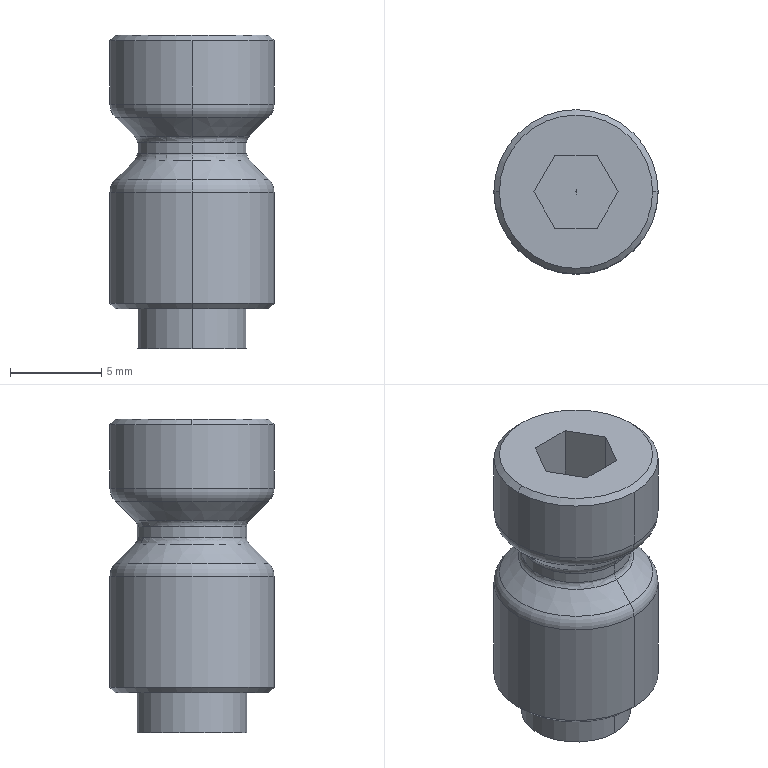Component | SolidWorks | GripperA3-2-1_SCHUNK-0303022-1 | 1 solid | 38 faces | box 9 x 9 x 17.2 mm | volume 756 mm3 | cylinder 10 | cone 10 | plane 10 | torus 8 | commonest cylinder face diameters 9 x4 6 x4 3.242 x2 | material 1.231 (40CrMnMoS8-6)
STEP:
#1=COLOUR_RGB('',0.7922,0.8196,0.9333);
#2=FILL_AREA_STYLE_COLOUR('',#1);
#3=FILL_AREA_STYLE('',(#2));
#4=SURFACE_STYLE_FILL_AREA(#3);
#5=SURFACE_SIDE_STYLE('',(#4));
#6=SURFACE_STYLE_USAGE(.BOTH.,#5);
#7=PRESENTATION_STYLE_ASSIGNMENT((#6));
#8=CARTESIAN_POINT('',(7.772,2.015,1.751));
#9=VERTEX_POINT('',#8);
#10=CARTESIAN_POINT('',(7.772,1.779,1.751));
#11=VERTEX_POINT('',#10);
#12=CARTESIAN_POINT('',(7.772,1.897,1.751));
#13=DIRECTION('',(0.,0.,1.));
#14=DIRECTION('',(0.,-1.,0.));
#15=AXIS2_PLACEMENT_3D('',#12,#13,#14);
#16=CIRCLE('',#15,0.1181);
#17=EDGE_CURVE('',#9,#11,#16,.T.);
#18=ORIENTED_EDGE('',*,*,#17,.F.);
#19=CARTESIAN_POINT('',(7.772,2.021,1.737));
#20=VERTEX_POINT('',#19);
#21=CARTESIAN_POINT('',(7.772,2.035,1.751));
#22=DIRECTION('',(1.,0.,-0.));
#23=DIRECTION('',(0.,0.,-1.));
#24=AXIS2_PLACEMENT_3D('',#21,#22,#23);
#25=CIRCLE('',#24,0.01969);
#26=EDGE_CURVE('',#9,#20,#25,.T.);
#27=ORIENTED_EDGE('',*,*,#26,.T.);
#28=CARTESIAN_POINT('',(7.772,1.773,1.737));
#29=VERTEX_POINT('',#28);
#30=CARTESIAN_POINT('',(7.772,1.897,1.737));
#31=DIRECTION('',(-0.,-0.,-1.));
#32=DIRECTION('',(0.,1.,0.));
#33=AXIS2_PLACEMENT_3D('',#30,#31,#32);
#34=CIRCLE('',#33,0.1239);
#35=EDGE_CURVE('',#29,#20,#34,.T.);
#36=ORIENTED_EDGE('',*,*,#35,.F.);
#37=CARTESIAN_POINT('',(7.772,1.759,1.751));
#38=DIRECTION('',(-1.,-0.,0.));
#39=DIRECTION('',(0.,0.,1.));
#40=AXIS2_PLACEMENT_3D('',#37,#38,#39);
#41=CIRCLE('',#40,0.01969);
#42=EDGE_CURVE('',#11,#29,#41,.T.);
#43=ORIENTED_EDGE('',*,*,#42,.F.);
#44=EDGE_LOOP('',(#18,#27,#36,#43));
#45=FACE_OUTER_BOUND('',#44,.T.);
#46=CARTESIAN_POINT('',(7.772,1.897,1.751));
#47=DIRECTION('',(0.,0.,1.));
#48=DIRECTION('',(-0.,-1.,0.));
#49=AXIS2_PLACEMENT_3D('',#46,#47,#48);
#50=TOROIDAL_SURFACE('',#49,0.1378,0.01969);
#51=ADVANCED_FACE('',(#45),#50,.F.);
#52=CARTESIAN_POINT('',(7.772,2.021,1.788));
#53=VERTEX_POINT('',#52);
#54=CARTESIAN_POINT('',(7.772,1.773,1.788));
#55=VERTEX_POINT('',#54);
#56=CARTESIAN_POINT('',(7.772,1.897,1.788));
#57=DIRECTION('',(0.,0.,1.));
#58=DIRECTION('',(0.,-1.,0.));
#59=AXIS2_PLACEMENT_3D('',#56,#57,#58);
#60=CIRCLE('',#59,0.1239);
#61=EDGE_CURVE('',#53,#55,#60,.T.);
#62=ORIENTED_EDGE('',*,*,#61,.F.);
#63=CARTESIAN_POINT('',(7.772,2.015,1.774));
#64=VERTEX_POINT('',#63);
#65=CARTESIAN_POINT('',(7.772,2.035,1.774));
#66=DIRECTION('',(1.,0.,-0.));
#67=DIRECTION('',(0.,0.,-1.));
#68=AXIS2_PLACEMENT_3D('',#65,#66,#67);
#69=CIRCLE('',#68,0.01969);
#70=EDGE_CURVE('',#53,#64,#69,.T.);
#71=ORIENTED_EDGE('',*,*,#70,.T.);
#72=CARTESIAN_POINT('',(7.772,1.779,1.774));
#73=VERTEX_POINT('',#72);
#74=CARTESIAN_POINT('',(7.772,1.897,1.774));
#75=DIRECTION('',(-0.,-0.,-1.));
#76=DIRECTION('',(0.,-1.,0.));
#77=AXIS2_PLACEMENT_3D('',#74,#75,#76);
#78=CIRCLE('',#77,0.1181);
#79=EDGE_CURVE('',#73,#64,#78,.T.);
#80=ORIENTED_EDGE('',*,*,#79,.F.);
#81=CARTESIAN_POINT('',(7.772,1.759,1.774));
#82=DIRECTION('',(-1.,-0.,0.));
#83=DIRECTION('',(0.,0.,1.));
#84=AXIS2_PLACEMENT_3D('',#81,#82,#83);
#85=CIRCLE('',#84,0.01969);
#86=EDGE_CURVE('',#55,#73,#85,.T.);
#87=ORIENTED_EDGE('',*,*,#86,.F.);
#88=EDGE_LOOP('',(#62,#71,#80,#87));
#89=FACE_OUTER_BOUND('',#88,.T.);
#90=CARTESIAN_POINT('',(7.772,1.897,1.774));
#91=DIRECTION('',(0.,0.,1.));
#92=DIRECTION('',(-0.,-1.,0.));
#93=AXIS2_PLACEMENT_3D('',#90,#91,#92);
#94=TOROIDAL_SURFACE('',#93,0.1378,0.01969);
#95=ADVANCED_FACE('',(#89),#94,.F.);
#96=CARTESIAN_POINT('',(7.772,2.074,1.668));
#97=VERTEX_POINT('',#96);
#98=CARTESIAN_POINT('',(7.772,1.72,1.668));
#99=VERTEX_POINT('',#98);
#100=CARTESIAN_POINT('',(7.772,1.897,1.668));
#101=DIRECTION('',(-0.,-0.,-1.));
#102=DIRECTION('',(-0.,-1.,0.));
#103=AXIS2_PLACEMENT_3D('',#100,#101,#102);
#104=CIRCLE('',#103,0.1772);
#105=EDGE_CURVE('',#97,#99,#104,.T.);
#106=ORIENTED_EDGE('',*,*,#105,.F.);
#107=CARTESIAN_POINT('',(7.772,2.063,1.695));
#108=VERTEX_POINT('',#107);
#109=CARTESIAN_POINT('',(7.772,2.035,1.668));
#110=DIRECTION('',(1.,0.,-0.));
#111=DIRECTION('',(0.,0.,-1.));
#112=AXIS2_PLACEMENT_3D('',#109,#110,#111);
#113=CIRCLE('',#112,0.03937);
#114=EDGE_CURVE('',#97,#108,#113,.T.);
#115=ORIENTED_EDGE('',*,*,#114,.T.);
#116=CARTESIAN_POINT('',(7.772,1.732,1.695));
#117=VERTEX_POINT('',#116);
#118=CARTESIAN_POINT('',(7.772,1.897,1.695));
#119=DIRECTION('',(0.,0.,1.));
#120=DIRECTION('',(0.,-1.,0.));
#121=AXIS2_PLACEMENT_3D('',#118,#119,#120);
#122=CIRCLE('',#121,0.1656);
#123=EDGE_CURVE('',#117,#108,#122,.T.);
#124=ORIENTED_EDGE('',*,*,#123,.F.);
#125=CARTESIAN_POINT('',(7.772,1.759,1.668));
#126=DIRECTION('',(-1.,-0.,0.));
#127=DIRECTION('',(0.,0.,1.));
#128=AXIS2_PLACEMENT_3D('',#125,#126,#127);
#129=CIRCLE('',#128,0.03937);
#130=EDGE_CURVE('',#99,#117,#129,.T.);
#131=ORIENTED_EDGE('',*,*,#130,.F.);
#132=EDGE_LOOP('',(#106,#115,#124,#131));
#133=FACE_OUTER_BOUND('',#132,.T.);
#134=CARTESIAN_POINT('',(7.772,1.897,1.668));
#135=DIRECTION('',(0.,0.,1.));
#136=DIRECTION('',(-0.,-1.,0.));
#137=AXIS2_PLACEMENT_3D('',#134,#135,#136);
#138=TOROIDAL_SURFACE('',#137,0.1378,0.03937);
#139=ADVANCED_FACE('',(#133),#138,.T.);
#140=CARTESIAN_POINT('',(7.772,1.72,1.858));
#141=VERTEX_POINT('',#140);
#142=CARTESIAN_POINT('',(7.772,2.074,1.858));
#143=VERTEX_POINT('',#142);
#144=CARTESIAN_POINT('',(7.772,1.897,1.858));
#145=DIRECTION('',(0.,0.,1.));
#146=DIRECTION('',(0.,1.,-0.));
#147=AXIS2_PLACEMENT_3D('',#144,#145,#146);
#148=CIRCLE('',#147,0.1772);
#149=EDGE_CURVE('',#141,#143,#148,.T.);
#150=ORIENTED_EDGE('',*,*,#149,.F.);
#151=CARTESIAN_POINT('',(7.772,1.732,1.83));
#152=VERTEX_POINT('',#151);
#153=CARTESIAN_POINT('',(7.772,1.759,1.858));
#154=DIRECTION('',(1.,0.,-0.));
#155=DIRECTION('',(0.,1.,0.));
#156=AXIS2_PLACEMENT_3D('',#153,#154,#155);
#157=CIRCLE('',#156,0.03937);
#158=EDGE_CURVE('',#141,#152,#157,.T.);
#159=ORIENTED_EDGE('',*,*,#158,.T.);
#160=CARTESIAN_POINT('',(7.772,2.063,1.83));
#161=VERTEX_POINT('',#160);
#162=CARTESIAN_POINT('',(7.772,1.897,1.83));
#163=DIRECTION('',(-0.,-0.,-1.));
#164=DIRECTION('',(0.,1.,-0.));
#165=AXIS2_PLACEMENT_3D('',#162,#163,#164);
#166=CIRCLE('',#165,0.1656);
#167=EDGE_CURVE('',#161,#152,#166,.T.);
#168=ORIENTED_EDGE('',*,*,#167,.F.);
#169=CARTESIAN_POINT('',(7.772,2.035,1.858));
#170=DIRECTION('',(-1.,-0.,0.));
#171=DIRECTION('',(0.,0.,1.));
#172=AXIS2_PLACEMENT_3D('',#169,#170,#171);
#173=CIRCLE('',#172,0.03937);
#174=EDGE_CURVE('',#143,#161,#173,.T.);
#175=ORIENTED_EDGE('',*,*,#174,.F.);
#176=EDGE_LOOP('',(#150,#159,#168,#175));
#177=FACE_OUTER_BOUND('',#176,.T.);
#178=CARTESIAN_POINT('',(7.772,1.897,1.858));
#179=DIRECTION('',(-0.,-0.,-1.));
#180=DIRECTION('',(0.,1.,-0.));
#181=AXIS2_PLACEMENT_3D('',#178,#179,#180);
#182=TOROIDAL_SURFACE('',#181,0.1378,0.03937);
#183=ADVANCED_FACE('',(#177),#182,.T.);
#184=CARTESIAN_POINT('',(7.95,1.897,1.995));
#185=VERTEX_POINT('',#184);
#186=CARTESIAN_POINT('',(7.772,1.72,1.995));
#187=VERTEX_POINT('',#186);
#188=CARTESIAN_POINT('',(7.772,1.897,1.995));
#189=DIRECTION('',(-0.,-0.,-1.));
#190=DIRECTION('',(0.,1.,-0.));
#191=AXIS2_PLACEMENT_3D('',#188,#189,#190);
#192=CIRCLE('',#191,0.1772);
#193=EDGE_CURVE('',#185,#187,#192,.T.);
#194=ORIENTED_EDGE('',*,*,#193,.T.);
#195=CARTESIAN_POINT('',(7.772,1.72,2.007));
#196=DIRECTION('',(-0.,-0.,-1.));
#197=VECTOR('',#196,39.37);
#198=LINE('',#195,#197);
#199=EDGE_CURVE('',#187,#141,#198,.T.);
#200=ORIENTED_EDGE('',*,*,#199,.T.);
#201=ORIENTED_EDGE('',*,*,#149,.T.);
#202=CARTESIAN_POINT('',(7.772,2.074,1.995));
#203=VERTEX_POINT('',#202);
#204=CARTESIAN_POINT('',(7.772,2.074,2.007));
#205=DIRECTION('',(-0.,-0.,-1.));
#206=VECTOR('',#205,39.37);
#207=LINE('',#204,#206);
#208=EDGE_CURVE('',#203,#143,#207,.T.);
#209=ORIENTED_EDGE('',*,*,#208,.F.);
#210=CARTESIAN_POINT('',(7.772,1.897,1.995));
#211=DIRECTION('',(-0.,-0.,-1.));
#212=DIRECTION('',(0.,1.,-0.));
#213=AXIS2_PLACEMENT_3D('',#210,#211,#212);
#214=CIRCLE('',#213,0.1772);
#215=EDGE_CURVE('',#203,#185,#214,.T.);
#216=ORIENTED_EDGE('',*,*,#215,.T.);
#217=EDGE_LOOP('',(#194,#200,#201,#209,#216));
#218=FACE_OUTER_BOUND('',#217,.T.);
#219=CARTESIAN_POINT('',(7.772,1.897,2.007));
#220=DIRECTION('',(-0.,-0.,-1.));
#221=DIRECTION('',(0.,1.,-0.));
#222=AXIS2_PLACEMENT_3D('',#219,#220,#221);
#223=CYLINDRICAL_SURFACE('',#222,0.1772);
#224=ADVANCED_FACE('',(#218),#223,.T.);
#225=CARTESIAN_POINT('',(7.607,1.897,2.007));
#226=VERTEX_POINT('',#225);
#227=CARTESIAN_POINT('',(7.938,1.897,2.007));
#228=VERTEX_POINT('',#227);
#229=CARTESIAN_POINT('',(7.772,1.897,2.007));
#230=DIRECTION('',(-0.,-0.,-1.));
#231=DIRECTION('',(-1.,-0.,0.));
#232=AXIS2_PLACEMENT_3D('',#229,#230,#231);
#233=CIRCLE('',#232,0.1654);
#234=EDGE_CURVE('',#226,#228,#233,.T.);
#235=ORIENTED_EDGE('',*,*,#234,.T.);
#236=CARTESIAN_POINT('',(7.95,1.897,1.995));
#237=DIRECTION('',(0.7071,0.,-0.7071));
#238=VECTOR('',#237,39.37);
#239=LINE('',#236,#238);
#240=EDGE_CURVE('',#228,#185,#239,.T.);
#241=ORIENTED_EDGE('',*,*,#240,.T.);
#242=ORIENTED_EDGE('',*,*,#215,.F.);
#243=CARTESIAN_POINT('',(7.595,1.897,1.995));
#244=VERTEX_POINT('',#243);
#245=CARTESIAN_POINT('',(7.772,1.897,1.995));
#246=DIRECTION('',(-0.,-0.,-1.));
#247=DIRECTION('',(0.,1.,-0.));
#248=AXIS2_PLACEMENT_3D('',#245,#246,#247);
#249=CIRCLE('',#248,0.1772);
#250=EDGE_CURVE('',#244,#203,#249,.T.);
#251=ORIENTED_EDGE('',*,*,#250,.F.);
#252=CARTESIAN_POINT('',(7.595,1.897,1.995));
#253=DIRECTION('',(-0.7071,-0.,-0.7071));
#254=VECTOR('',#253,39.37);
#255=LINE('',#252,#254);
#256=EDGE_CURVE('',#226,#244,#255,.T.);
#257=ORIENTED_EDGE('',*,*,#256,.F.);
#258=EDGE_LOOP('',(#235,#241,#242,#251,#257));
#259=FACE_OUTER_BOUND('',#258,.T.);
#260=CARTESIAN_POINT('',(7.772,1.897,1.995));
#261=DIRECTION('',(-0.,-0.,-1.));
#262=DIRECTION('',(-1.,-0.,0.));
#263=AXIS2_PLACEMENT_3D('',#260,#261,#262);
#264=CONICAL_SURFACE('',#263,0.1772,0.7854);
#265=ADVANCED_FACE('',(#259),#264,.T.);
#266=CARTESIAN_POINT('',(7.772,1.897,1.788));
#267=DIRECTION('',(0.,0.,1.));
#268=DIRECTION('',(0.,-1.,0.));
#269=AXIS2_PLACEMENT_3D('',#266,#267,#268);
#270=CIRCLE('',#269,0.1239);
#271=EDGE_CURVE('',#55,#53,#270,.T.);
#272=ORIENTED_EDGE('',*,*,#271,.T.);
#273=CARTESIAN_POINT('',(7.772,2.103,1.87));
#274=DIRECTION('',(0.,0.7071,0.7071));
#275=VECTOR('',#274,39.37);
#276=LINE('',#273,#275);
#277=EDGE_CURVE('',#53,#161,#276,.T.);
#278=ORIENTED_EDGE('',*,*,#277,.T.);
#279=ORIENTED_EDGE('',*,*,#167,.T.);
#280=CARTESIAN_POINT('',(7.772,1.691,1.87));
#281=DIRECTION('',(0.,-0.7071,0.7071));
#282=VECTOR('',#281,39.37);
#283=LINE('',#280,#282);
#284=EDGE_CURVE('',#55,#152,#283,.T.);
#285=ORIENTED_EDGE('',*,*,#284,.F.);
#286=EDGE_LOOP('',(#272,#278,#279,#285));
#287=FACE_OUTER_BOUND('',#286,.T.);
#288=CARTESIAN_POINT('',(7.772,1.897,1.87));
#289=DIRECTION('',(0.,0.,1.));
#290=DIRECTION('',(0.,-1.,0.));
#291=AXIS2_PLACEMENT_3D('',#288,#289,#290);
#292=CONICAL_SURFACE('',#291,0.2058,0.7854);
#293=ADVANCED_FACE('',(#287),#292,.T.);
#294=CARTESIAN_POINT('',(7.772,1.897,1.751));
#295=DIRECTION('',(0.,0.,1.));
#296=DIRECTION('',(0.,-1.,0.));
#297=AXIS2_PLACEMENT_3D('',#294,#295,#296);
#298=CIRCLE('',#297,0.1181);
#299=EDGE_CURVE('',#11,#9,#298,.T.);
#300=ORIENTED_EDGE('',*,*,#299,.T.);
#301=CARTESIAN_POINT('',(7.772,2.015,1.772));
#302=DIRECTION('',(0.,0.,1.));
#303=VECTOR('',#302,39.37);
#304=LINE('',#301,#303);
#305=EDGE_CURVE('',#9,#64,#304,.T.);
#306=ORIENTED_EDGE('',*,*,#305,.T.);
#307=CARTESIAN_POINT('',(7.772,1.897,1.774));
#308=DIRECTION('',(-0.,-0.,-1.));
#309=DIRECTION('',(0.,-1.,0.));
#310=AXIS2_PLACEMENT_3D('',#307,#308,#309);
#311=CIRCLE('',#310,0.1181);
#312=EDGE_CURVE('',#64,#73,#311,.T.);
#313=ORIENTED_EDGE('',*,*,#312,.T.);
#314=CARTESIAN_POINT('',(7.772,1.779,1.772));
#315=DIRECTION('',(0.,0.,1.));
#316=VECTOR('',#315,39.37);
#317=LINE('',#314,#316);
#318=EDGE_CURVE('',#11,#73,#317,.T.);
#319=ORIENTED_EDGE('',*,*,#318,.F.);
#320=EDGE_LOOP('',(#300,#306,#313,#319));
#321=FACE_OUTER_BOUND('',#320,.T.);
#322=CARTESIAN_POINT('',(7.772,1.897,1.772));
#323=DIRECTION('',(0.,0.,1.));
#324=DIRECTION('',(0.,-1.,0.));
#325=AXIS2_PLACEMENT_3D('',#322,#323,#324);
#326=CYLINDRICAL_SURFACE('',#325,0.1181);
#327=ADVANCED_FACE('',(#321),#326,.T.);
#328=CARTESIAN_POINT('',(7.772,1.897,1.737));
#329=DIRECTION('',(-0.,-0.,-1.));
#330=DIRECTION('',(0.,1.,0.));
#331=AXIS2_PLACEMENT_3D('',#328,#329,#330);
#332=CIRCLE('',#331,0.1239);
#333=EDGE_CURVE('',#20,#29,#332,.T.);
#334=ORIENTED_EDGE('',*,*,#333,.T.);
#335=CARTESIAN_POINT('',(7.772,1.779,1.743));
#336=DIRECTION('',(0.,-0.7071,-0.7071));
#337=VECTOR('',#336,39.37);
#338=LINE('',#335,#337);
#339=EDGE_CURVE('',#29,#117,#338,.T.);
#340=ORIENTED_EDGE('',*,*,#339,.T.);
#341=ORIENTED_EDGE('',*,*,#123,.T.);
#342=CARTESIAN_POINT('',(7.772,2.015,1.743));
#343=DIRECTION('',(-0.,0.7071,-0.7071));
#344=VECTOR('',#343,39.37);
#345=LINE('',#342,#344);
#346=EDGE_CURVE('',#20,#108,#345,.T.);
#347=ORIENTED_EDGE('',*,*,#346,.F.);
#348=EDGE_LOOP('',(#334,#340,#341,#347));
#349=FACE_OUTER_BOUND('',#348,.T.);
#350=CARTESIAN_POINT('',(7.772,1.897,1.743));
#351=DIRECTION('',(-0.,-0.,-1.));
#352=DIRECTION('',(0.,1.,0.));
#353=AXIS2_PLACEMENT_3D('',#350,#351,#352);
#354=CONICAL_SURFACE('',#353,0.1181,0.7854);
#355=ADVANCED_FACE('',(#349),#354,.T.);
#356=CARTESIAN_POINT('',(7.772,1.732,1.416));
#357=VERTEX_POINT('',#356);
#358=CARTESIAN_POINT('',(7.772,2.063,1.416));
#359=VERTEX_POINT('',#358);
#360=CARTESIAN_POINT('',(7.772,1.897,1.416));
#361=DIRECTION('',(0.,0.,1.));
#362=DIRECTION('',(0.,-1.,0.));
#363=AXIS2_PLACEMENT_3D('',#360,#361,#362);
#364=CIRCLE('',#363,0.1654);
#365=EDGE_CURVE('',#357,#359,#364,.T.);
#366=ORIENTED_EDGE('',*,*,#365,.T.);
#367=CARTESIAN_POINT('',(7.772,2.074,1.428));
#368=VERTEX_POINT('',#367);
#369=CARTESIAN_POINT('',(7.772,2.074,1.428));
#370=DIRECTION('',(0.,0.7071,0.7071));
#371=VECTOR('',#370,39.37);
#372=LINE('',#369,#371);
#373=EDGE_CURVE('',#359,#368,#372,.T.);
#374=ORIENTED_EDGE('',*,*,#373,.T.);
#375=CARTESIAN_POINT('',(7.772,1.72,1.428));
#376=VERTEX_POINT('',#375);
#377=CARTESIAN_POINT('',(7.772,1.897,1.428));
#378=DIRECTION('',(0.,0.,1.));
#379=DIRECTION('',(-0.,1.,-0.));
#380=AXIS2_PLACEMENT_3D('',#377,#378,#379);
#381=CIRCLE('',#380,0.1772);
#382=EDGE_CURVE('',#376,#368,#381,.T.);
#383=ORIENTED_EDGE('',*,*,#382,.F.);
#384=CARTESIAN_POINT('',(7.772,1.72,1.428));
#385=DIRECTION('',(0.,-0.7071,0.7071));
#386=VECTOR('',#385,39.37);
#387=LINE('',#384,#386);
#388=EDGE_CURVE('',#357,#376,#387,.T.);
#389=ORIENTED_EDGE('',*,*,#388,.F.);
#390=EDGE_LOOP('',(#366,#374,#383,#389));
#391=FACE_OUTER_BOUND('',#390,.T.);
#392=CARTESIAN_POINT('',(7.772,1.897,1.428));
#393=DIRECTION('',(0.,0.,1.));
#394=DIRECTION('',(0.,-1.,0.));
#395=AXIS2_PLACEMENT_3D('',#392,#393,#394);
#396=CONICAL_SURFACE('',#395,0.1772,0.7854);
#397=ADVANCED_FACE('',(#391),#396,.T.);
#398=CARTESIAN_POINT('',(7.772,2.015,1.416));
#399=VERTEX_POINT('',#398);
#400=CARTESIAN_POINT('',(7.772,1.779,1.416));
#401=VERTEX_POINT('',#400);
#402=CARTESIAN_POINT('',(7.772,1.897,1.416));
#403=DIRECTION('',(-0.,-0.,-1.));
#404=DIRECTION('',(0.,1.,0.));
#405=AXIS2_PLACEMENT_3D('',#402,#403,#404);
#406=CIRCLE('',#405,0.1181);
#407=EDGE_CURVE('',#399,#401,#406,.T.);
#408=ORIENTED_EDGE('',*,*,#407,.T.);
#409=CARTESIAN_POINT('',(7.772,1.779,1.33));
#410=VERTEX_POINT('',#409);
#411=CARTESIAN_POINT('',(7.772,1.779,2.007));
#412=DIRECTION('',(-0.,-0.,-1.));
#413=VECTOR('',#412,39.37);
#414=LINE('',#411,#413);
#415=EDGE_CURVE('',#401,#410,#414,.T.);
#416=ORIENTED_EDGE('',*,*,#415,.T.);
#417=CARTESIAN_POINT('',(7.772,2.015,1.33));
#418=VERTEX_POINT('',#417);
#419=CARTESIAN_POINT('',(7.772,1.897,1.33));
#420=DIRECTION('',(0.,0.,1.));
#421=DIRECTION('',(0.,1.,0.));
#422=AXIS2_PLACEMENT_3D('',#419,#420,#421);
#423=CIRCLE('',#422,0.1181);
#424=EDGE_CURVE('',#410,#418,#423,.T.);
#425=ORIENTED_EDGE('',*,*,#424,.T.);
#426=CARTESIAN_POINT('',(7.772,2.015,2.007));
#427=DIRECTION('',(-0.,-0.,-1.));
#428=VECTOR('',#427,39.37);
#429=LINE('',#426,#428);
#430=EDGE_CURVE('',#399,#418,#429,.T.);
#431=ORIENTED_EDGE('',*,*,#430,.F.);
#432=EDGE_LOOP('',(#408,#416,#425,#431));
#433=FACE_OUTER_BOUND('',#432,.T.);
#434=CARTESIAN_POINT('',(7.772,1.897,2.007));
#435=DIRECTION('',(-0.,-0.,-1.));
#436=DIRECTION('',(0.,1.,0.));
#437=AXIS2_PLACEMENT_3D('',#434,#435,#436);
#438=CYLINDRICAL_SURFACE('',#437,0.1181);
#439=ADVANCED_FACE('',(#433),#438,.T.);
#440=CARTESIAN_POINT('',(7.772,1.833,1.772));
#441=VERTEX_POINT('',#440);
#442=CARTESIAN_POINT('',(7.772,1.961,1.772));
#443=VERTEX_POINT('',#442);
#444=CARTESIAN_POINT('',(7.772,1.897,1.772));
#445=DIRECTION('',(-0.,-0.,-1.));
#446=DIRECTION('',(0.,1.,0.));
#447=AXIS2_PLACEMENT_3D('',#444,#445,#446);
#448=CIRCLE('',#447,0.06382);
#449=EDGE_CURVE('',#441,#443,#448,.T.);
#450=ORIENTED_EDGE('',*,*,#449,.F.);
#451=CARTESIAN_POINT('',(7.772,1.833,1.33));
#452=VERTEX_POINT('',#451);
#453=CARTESIAN_POINT('',(7.772,1.833,2.007));
#454=DIRECTION('',(-0.,-0.,-1.));
#455=VECTOR('',#454,39.37);
#456=LINE('',#453,#455);
#457=EDGE_CURVE('',#441,#452,#456,.T.);
#458=ORIENTED_EDGE('',*,*,#457,.T.);
#459=CARTESIAN_POINT('',(7.772,1.961,1.33));
#460=VERTEX_POINT('',#459);
#461=CARTESIAN_POINT('',(7.772,1.897,1.33));
#462=DIRECTION('',(-0.,-0.,-1.));
#463=DIRECTION('',(0.,1.,0.));
#464=AXIS2_PLACEMENT_3D('',#461,#462,#463);
#465=CIRCLE('',#464,0.06382);
#466=EDGE_CURVE('',#452,#460,#465,.T.);
#467=ORIENTED_EDGE('',*,*,#466,.T.);
#468=CARTESIAN_POINT('',(7.772,1.961,2.007));
#469=DIRECTION('',(-0.,-0.,-1.));
#470=VECTOR('',#469,39.37);
#471=LINE('',#468,#470);
#472=EDGE_CURVE('',#443,#460,#471,.T.);
#473=ORIENTED_EDGE('',*,*,#472,.F.);
#474=EDGE_LOOP('',(#450,#458,#467,#473));
#475=FACE_OUTER_BOUND('',#474,.T.);
#476=CARTESIAN_POINT('',(7.772,1.897,2.007));
#477=DIRECTION('',(-0.,-0.,-1.));
#478=DIRECTION('',(0.,1.,0.));
#479=AXIS2_PLACEMENT_3D('',#476,#477,#478);
#480=CYLINDRICAL_SURFACE('',#479,0.06382);
#481=ADVANCED_FACE('',(#475),#480,.F.);
#482=ORIENTED_EDGE('',*,*,#105,.T.);
#483=CARTESIAN_POINT('',(7.772,1.72,2.007));
#484=DIRECTION('',(-0.,-0.,-1.));
#485=VECTOR('',#484,39.37);
#486=LINE('',#483,#485);
#487=EDGE_CURVE('',#99,#376,#486,.T.);
#488=ORIENTED_EDGE('',*,*,#487,.T.);
#489=ORIENTED_EDGE('',*,*,#382,.T.);
#490=CARTESIAN_POINT('',(7.772,2.074,2.007));
#491=DIRECTION('',(-0.,-0.,-1.));
#492=VECTOR('',#491,39.37);
#493=LINE('',#490,#492);
#494=EDGE_CURVE('',#97,#368,#493,.T.);
#495=ORIENTED_EDGE('',*,*,#494,.F.);
#496=EDGE_LOOP('',(#482,#488,#489,#495));
#497=FACE_OUTER_BOUND('',#496,.T.);
#498=CARTESIAN_POINT('',(7.772,1.897,2.007));
#499=DIRECTION('',(-0.,-0.,-1.));
#500=DIRECTION('',(0.,1.,-0.));
#501=AXIS2_PLACEMENT_3D('',#498,#499,#500);
#502=CYLINDRICAL_SURFACE('',#501,0.1772);
#503=ADVANCED_FACE('',(#497),#502,.T.);
#504=CARTESIAN_POINT('',(7.772,1.897,1.81));
#505=VERTEX_POINT('',#504);
#506=CARTESIAN_POINT('',(7.772,1.897,1.81));
#507=VERTEX_POINT('',#506);
#508=CARTESIAN_POINT('',(7.772,1.897,1.81));
#509=DIRECTION('',(-0.,-0.,-1.));
#510=DIRECTION('',(0.,-1.,0.));
#511=AXIS2_PLACEMENT_3D('',#508,#509,#510);
#512=CIRCLE('',#511,0.0001128);
#513=EDGE_CURVE('',#505,#507,#512,.T.);
#514=ORIENTED_EDGE('',*,*,#513,.F.);
#515=CARTESIAN_POINT('',(7.772,1.833,1.772));
#516=DIRECTION('',(0.,-0.8572,-0.515));
#517=VECTOR('',#516,39.37);
#518=LINE('',#515,#517);
#519=EDGE_CURVE('',#505,#441,#518,.T.);
#520=ORIENTED_EDGE('',*,*,#519,.T.);
#521=ORIENTED_EDGE('',*,*,#449,.T.);
#522=CARTESIAN_POINT('',(7.772,1.961,1.772));
#523=DIRECTION('',(-0.,0.8572,-0.515));
#524=VECTOR('',#523,39.37);
#525=LINE('',#522,#524);
#526=EDGE_CURVE('',#507,#443,#525,.T.);
#527=ORIENTED_EDGE('',*,*,#526,.F.);
#528=EDGE_LOOP('',(#514,#520,#521,#527));
#529=FACE_OUTER_BOUND('',#528,.T.);
#530=CARTESIAN_POINT('',(7.772,1.897,1.772));
#531=DIRECTION('',(-0.,-0.,-1.));
#532=DIRECTION('',(0.,1.,0.));
#533=AXIS2_PLACEMENT_3D('',#530,#531,#532);
#534=CONICAL_SURFACE('',#533,0.06382,1.03);
#535=ADVANCED_FACE('',(#529),#534,.F.);
#536=ORIENTED_EDGE('',*,*,#519,.F.);
#537=CARTESIAN_POINT('',(7.772,1.897,1.81));
#538=DIRECTION('',(-0.,-0.,-1.));
#539=DIRECTION('',(0.,-1.,0.));
#540=AXIS2_PLACEMENT_3D('',#537,#538,#539);
#541=CIRCLE('',#540,0.0001128);
#542=EDGE_CURVE('',#507,#505,#541,.T.);
#543=ORIENTED_EDGE('',*,*,#542,.F.);
#544=ORIENTED_EDGE('',*,*,#526,.T.);
#545=CARTESIAN_POINT('',(7.772,1.897,1.772));
#546=DIRECTION('',(-0.,-0.,-1.));
#547=DIRECTION('',(0.,1.,0.));
#548=AXIS2_PLACEMENT_3D('',#545,#546,#547);
#549=CIRCLE('',#548,0.06382);
#550=EDGE_CURVE('',#443,#441,#549,.T.);
#551=ORIENTED_EDGE('',*,*,#550,.T.);
#552=EDGE_LOOP('',(#536,#543,#544,#551));
#553=FACE_OUTER_BOUND('',#552,.T.);
#554=CARTESIAN_POINT('',(7.772,1.897,1.772));
#555=DIRECTION('',(-0.,-0.,-1.));
#556=DIRECTION('',(0.,1.,0.));
#557=AXIS2_PLACEMENT_3D('',#554,#555,#556);
#558=CONICAL_SURFACE('',#557,0.06382,1.03);
#559=ADVANCED_FACE('',(#553),#558,.F.);
#560=ORIENTED_EDGE('',*,*,#487,.F.);
#561=CARTESIAN_POINT('',(7.772,1.897,1.668));
#562=DIRECTION('',(-0.,-0.,-1.));
#563=DIRECTION('',(0.,-1.,0.));
#564=AXIS2_PLACEMENT_3D('',#561,#562,#563);
#565=CIRCLE('',#564,0.1772);
#566=EDGE_CURVE('',#99,#97,#565,.T.);
#567=ORIENTED_EDGE('',*,*,#566,.T.);
#568=ORIENTED_EDGE('',*,*,#494,.T.);
#569=CARTESIAN_POINT('',(7.772,1.897,1.428));
#570=DIRECTION('',(0.,0.,1.));
#571=DIRECTION('',(0.,1.,-0.));
#572=AXIS2_PLACEMENT_3D('',#569,#570,#571);
#573=CIRCLE('',#572,0.1772);
#574=EDGE_CURVE('',#368,#376,#573,.T.);
#575=ORIENTED_EDGE('',*,*,#574,.T.);
#576=EDGE_LOOP('',(#560,#567,#568,#575));
#577=FACE_OUTER_BOUND('',#576,.T.);
#578=CARTESIAN_POINT('',(7.772,1.897,2.007));
#579=DIRECTION('',(-0.,-0.,-1.));
#580=DIRECTION('',(0.,1.,-0.));
#581=AXIS2_PLACEMENT_3D('',#578,#579,#580);
#582=CYLINDRICAL_SURFACE('',#581,0.1772);
#583=ADVANCED_FACE('',(#577),#582,.T.);
#584=ORIENTED_EDGE('',*,*,#373,.F.);
#585=CARTESIAN_POINT('',(7.772,1.897,1.416));
#586=DIRECTION('',(0.,0.,1.));
#587=DIRECTION('',(0.,-1.,0.));
#588=AXIS2_PLACEMENT_3D('',#585,#586,#587);
#589=CIRCLE('',#588,0.1654);
#590=EDGE_CURVE('',#359,#357,#589,.T.);
#591=ORIENTED_EDGE('',*,*,#590,.T.);
#592=ORIENTED_EDGE('',*,*,#388,.T.);
#593=ORIENTED_EDGE('',*,*,#574,.F.);
#594=EDGE_LOOP('',(#584,#591,#592,#593));
#595=FACE_OUTER_BOUND('',#594,.T.);
#596=CARTESIAN_POINT('',(7.772,1.897,1.428));
#597=DIRECTION('',(0.,0.,1.));
#598=DIRECTION('',(0.,-1.,0.));
#599=AXIS2_PLACEMENT_3D('',#596,#597,#598);
#600=CONICAL_SURFACE('',#599,0.1772,0.7854);
#601=ADVANCED_FACE('',(#595),#600,.T.);
#602=ORIENTED_EDGE('',*,*,#407,.F.);
#603=CARTESIAN_POINT('',(7.772,1.897,1.416));
#604=DIRECTION('',(-0.,-0.,-1.));
#605=DIRECTION('',(0.,1.,0.));
#606=AXIS2_PLACEMENT_3D('',#603,#604,#605);
#607=CIRCLE('',#606,0.1181);
#608=EDGE_CURVE('',#401,#399,#607,.T.);
#609=ORIENTED_EDGE('',*,*,#608,.F.);
#610=EDGE_LOOP('',(#602,#609));
#611=FACE_BOUND('',#610,.T.);
#612=ORIENTED_EDGE('',*,*,#365,.F.);
#613=ORIENTED_EDGE('',*,*,#590,.F.);
#614=EDGE_LOOP('',(#612,#613));
#615=FACE_OUTER_BOUND('',#614,.T.);
#616=CARTESIAN_POINT('',(7.772,1.779,1.416));
#617=DIRECTION('',(0.,0.,1.));
#618=DIRECTION('',(0.,-1.,0.));
#619=AXIS2_PLACEMENT_3D('',#616,#617,#618);
#620=PLANE('',#619);
#621=ADVANCED_FACE('',(#611,#615),#620,.F.);
#622=ORIENTED_EDGE('',*,*,#415,.F.);
#623=ORIENTED_EDGE('',*,*,#608,.T.);
#624=ORIENTED_EDGE('',*,*,#430,.T.);
#625=CARTESIAN_POINT('',(7.772,1.897,1.33));
#626=DIRECTION('',(0.,0.,1.));
#627=DIRECTION('',(0.,1.,0.));
#628=AXIS2_PLACEMENT_3D('',#625,#626,#627);
#629=CIRCLE('',#628,0.1181);
#630=EDGE_CURVE('',#418,#410,#629,.T.);
#631=ORIENTED_EDGE('',*,*,#630,.T.);
#632=EDGE_LOOP('',(#622,#623,#624,#631));
#633=FACE_OUTER_BOUND('',#632,.T.);
#634=CARTESIAN_POINT('',(7.772,1.897,2.007));
#635=DIRECTION('',(-0.,-0.,-1.));
#636=DIRECTION('',(0.,1.,0.));
#637=AXIS2_PLACEMENT_3D('',#634,#635,#636);
#638=CYLINDRICAL_SURFACE('',#637,0.1181);
#639=ADVANCED_FACE('',(#633),#638,.T.);
#640=CARTESIAN_POINT('',(7.772,1.897,1.33));
#641=DIRECTION('',(-0.,-0.,-1.));
#642=DIRECTION('',(0.,1.,0.));
#643=AXIS2_PLACEMENT_3D('',#640,#641,#642);
#644=CIRCLE('',#643,0.06382);
#645=EDGE_CURVE('',#460,#452,#644,.T.);
#646=ORIENTED_EDGE('',*,*,#645,.F.);
#647=ORIENTED_EDGE('',*,*,#466,.F.);
#648=EDGE_LOOP('',(#646,#647));
#649=FACE_BOUND('',#648,.T.);
#650=ORIENTED_EDGE('',*,*,#630,.F.);
#651=ORIENTED_EDGE('',*,*,#424,.F.);
#652=EDGE_LOOP('',(#650,#651));
#653=FACE_OUTER_BOUND('',#652,.T.);
#654=CARTESIAN_POINT('',(7.772,1.833,1.33));
#655=DIRECTION('',(0.,0.,1.));
#656=DIRECTION('',(0.,-1.,0.));
#657=AXIS2_PLACEMENT_3D('',#654,#655,#656);
#658=PLANE('',#657);
#659=ADVANCED_FACE('',(#649,#653),#658,.F.);
#660=ORIENTED_EDGE('',*,*,#457,.F.);
#661=ORIENTED_EDGE('',*,*,#550,.F.);
#662=ORIENTED_EDGE('',*,*,#472,.T.);
#663=ORIENTED_EDGE('',*,*,#645,.T.);
#664=EDGE_LOOP('',(#660,#661,#662,#663));
#665=FACE_OUTER_BOUND('',#664,.T.);
#666=CARTESIAN_POINT('',(7.772,1.897,2.007));
#667=DIRECTION('',(-0.,-0.,-1.));
#668=DIRECTION('',(0.,1.,0.));
#669=AXIS2_PLACEMENT_3D('',#666,#667,#668);
#670=CYLINDRICAL_SURFACE('',#669,0.06382);
#671=ADVANCED_FACE('',(#665),#670,.F.);
#672=ORIENTED_EDGE('',*,*,#339,.F.);
#673=ORIENTED_EDGE('',*,*,#35,.T.);
#674=ORIENTED_EDGE('',*,*,#346,.T.);
#675=CARTESIAN_POINT('',(7.772,1.897,1.695));
#676=DIRECTION('',(0.,0.,1.));
#677=DIRECTION('',(0.,-1.,0.));
#678=AXIS2_PLACEMENT_3D('',#675,#676,#677);
#679=CIRCLE('',#678,0.1656);
#680=EDGE_CURVE('',#108,#117,#679,.T.);
#681=ORIENTED_EDGE('',*,*,#680,.T.);
#682=EDGE_LOOP('',(#672,#673,#674,#681));
#683=FACE_OUTER_BOUND('',#682,.T.);
#684=CARTESIAN_POINT('',(7.772,1.897,1.743));
#685=DIRECTION('',(-0.,-0.,-1.));
#686=DIRECTION('',(0.,1.,0.));
#687=AXIS2_PLACEMENT_3D('',#684,#685,#686);
#688=CONICAL_SURFACE('',#687,0.1181,0.7854);
#689=ADVANCED_FACE('',(#683),#688,.T.);
#690=ORIENTED_EDGE('',*,*,#305,.F.);
#691=ORIENTED_EDGE('',*,*,#17,.T.);
#692=ORIENTED_EDGE('',*,*,#318,.T.);
#693=ORIENTED_EDGE('',*,*,#79,.T.);
#694=EDGE_LOOP('',(#690,#691,#692,#693));
#695=FACE_OUTER_BOUND('',#694,.T.);
#696=CARTESIAN_POINT('',(7.772,1.897,1.772));
#697=DIRECTION('',(0.,0.,1.));
#698=DIRECTION('',(0.,-1.,0.));
#699=AXIS2_PLACEMENT_3D('',#696,#697,#698);
#700=CYLINDRICAL_SURFACE('',#699,0.1181);
#701=ADVANCED_FACE('',(#695),#700,.T.);
#702=ORIENTED_EDGE('',*,*,#277,.F.);
#703=ORIENTED_EDGE('',*,*,#61,.T.);
#704=ORIENTED_EDGE('',*,*,#284,.T.);
#705=CARTESIAN_POINT('',(7.772,1.897,1.83));
#706=DIRECTION('',(-0.,-0.,-1.));
#707=DIRECTION('',(0.,1.,-0.));
#708=AXIS2_PLACEMENT_3D('',#705,#706,#707);
#709=CIRCLE('',#708,0.1656);
#710=EDGE_CURVE('',#152,#161,#709,.T.);
#711=ORIENTED_EDGE('',*,*,#710,.T.);
#712=EDGE_LOOP('',(#702,#703,#704,#711));
#713=FACE_OUTER_BOUND('',#712,.T.);
#714=CARTESIAN_POINT('',(7.772,1.897,1.87));
#715=DIRECTION('',(0.,0.,1.));
#716=DIRECTION('',(0.,-1.,0.));
#717=AXIS2_PLACEMENT_3D('',#714,#715,#716);
#718=CONICAL_SURFACE('',#717,0.2058,0.7854);
#719=ADVANCED_FACE('',(#713),#718,.T.);
#720=CARTESIAN_POINT('',(7.682,1.897,2.007));
#721=VERTEX_POINT('',#720);
#722=CARTESIAN_POINT('',(7.727,1.818,2.007));
#723=VERTEX_POINT('',#722);
#724=CARTESIAN_POINT('',(7.682,1.897,2.007));
#725=DIRECTION('',(0.5,-0.866,0.));
#726=VECTOR('',#725,39.37);
#727=LINE('',#724,#726);
#728=EDGE_CURVE('',#721,#723,#727,.T.);
#729=ORIENTED_EDGE('',*,*,#728,.F.);
#730=CARTESIAN_POINT('',(7.727,1.976,2.007));
#731=VERTEX_POINT('',#730);
#732=CARTESIAN_POINT('',(7.727,1.976,2.007));
#733=DIRECTION('',(-0.5,-0.866,0.));
#734=VECTOR('',#733,39.37);
#735=LINE('',#732,#734);
#736=EDGE_CURVE('',#731,#721,#735,.T.);
#737=ORIENTED_EDGE('',*,*,#736,.F.);
#738=CARTESIAN_POINT('',(7.818,1.976,2.007));
#739=VERTEX_POINT('',#738);
#740=CARTESIAN_POINT('',(7.818,1.976,2.007));
#741=DIRECTION('',(-1.,-0.,0.));
#742=VECTOR('',#741,39.37);
#743=LINE('',#740,#742);
#744=EDGE_CURVE('',#739,#731,#743,.T.);
#745=ORIENTED_EDGE('',*,*,#744,.F.);
#746=CARTESIAN_POINT('',(7.863,1.897,2.007));
#747=VERTEX_POINT('',#746);
#748=CARTESIAN_POINT('',(7.863,1.897,2.007));
#749=DIRECTION('',(-0.5,0.866,-0.));
#750=VECTOR('',#749,39.37);
#751=LINE('',#748,#750);
#752=EDGE_CURVE('',#747,#739,#751,.T.);
#753=ORIENTED_EDGE('',*,*,#752,.F.);
#754=CARTESIAN_POINT('',(7.818,1.818,2.007));
#755=VERTEX_POINT('',#754);
#756=CARTESIAN_POINT('',(7.818,1.818,2.007));
#757=DIRECTION('',(0.5,0.866,-0.));
#758=VECTOR('',#757,39.37);
#759=LINE('',#756,#758);
#760=EDGE_CURVE('',#755,#747,#759,.T.);
#761=ORIENTED_EDGE('',*,*,#760,.F.);
#762=CARTESIAN_POINT('',(7.727,1.818,2.007));
#763=DIRECTION('',(1.,0.,-0.));
#764=VECTOR('',#763,39.37);
#765=LINE('',#762,#764);
#766=EDGE_CURVE('',#723,#755,#765,.T.);
#767=ORIENTED_EDGE('',*,*,#766,.F.);
#768=EDGE_LOOP('',(#729,#737,#745,#753,#761,#767));
#769=FACE_BOUND('',#768,.T.);
#770=ORIENTED_EDGE('',*,*,#234,.F.);
#771=CARTESIAN_POINT('',(7.772,1.897,2.007));
#772=DIRECTION('',(-0.,-0.,-1.));
#773=DIRECTION('',(-1.,-0.,0.));
#774=AXIS2_PLACEMENT_3D('',#771,#772,#773);
#775=CIRCLE('',#774,0.1654);
#776=EDGE_CURVE('',#228,#226,#775,.T.);
#777=ORIENTED_EDGE('',*,*,#776,.F.);
#778=EDGE_LOOP('',(#770,#777));
#779=FACE_OUTER_BOUND('',#778,.T.);
#780=CARTESIAN_POINT('',(7.772,1.732,2.007));
#781=DIRECTION('',(-0.,-0.,-1.));
#782=DIRECTION('',(-0.,1.,-0.));
#783=AXIS2_PLACEMENT_3D('',#780,#781,#782);
#784=PLANE('',#783);
#785=ADVANCED_FACE('',(#769,#779),#784,.F.);
#786=ORIENTED_EDGE('',*,*,#240,.F.);
#787=ORIENTED_EDGE('',*,*,#776,.T.);
#788=ORIENTED_EDGE('',*,*,#256,.T.);
#789=CARTESIAN_POINT('',(7.772,1.897,1.995));
#790=DIRECTION('',(-0.,-0.,-1.));
#791=DIRECTION('',(0.,1.,-0.));
#792=AXIS2_PLACEMENT_3D('',#789,#790,#791);
#793=CIRCLE('',#792,0.1772);
#794=EDGE_CURVE('',#187,#244,#793,.T.);
#795=ORIENTED_EDGE('',*,*,#794,.F.);
#796=ORIENTED_EDGE('',*,*,#193,.F.);
#797=EDGE_LOOP('',(#786,#787,#788,#795,#796));
#798=FACE_OUTER_BOUND('',#797,.T.);
#799=CARTESIAN_POINT('',(7.772,1.897,1.995));
#800=DIRECTION('',(-0.,-0.,-1.));
#801=DIRECTION('',(-1.,-0.,0.));
#802=AXIS2_PLACEMENT_3D('',#799,#800,#801);
#803=CONICAL_SURFACE('',#802,0.1772,0.7854);
#804=ADVANCED_FACE('',(#798),#803,.T.);
#805=ORIENTED_EDGE('',*,*,#199,.F.);
#806=ORIENTED_EDGE('',*,*,#794,.T.);
#807=ORIENTED_EDGE('',*,*,#250,.T.);
#808=ORIENTED_EDGE('',*,*,#208,.T.);
#809=CARTESIAN_POINT('',(7.772,1.897,1.858));
#810=DIRECTION('',(0.,0.,1.));
#811=DIRECTION('',(0.,1.,-0.));
#812=AXIS2_PLACEMENT_3D('',#809,#810,#811);
#813=CIRCLE('',#812,0.1772);
#814=EDGE_CURVE('',#143,#141,#813,.T.);
#815=ORIENTED_EDGE('',*,*,#814,.T.);
#816=EDGE_LOOP('',(#805,#806,#807,#808,#815));
#817=FACE_OUTER_BOUND('',#816,.T.);
#818=CARTESIAN_POINT('',(7.772,1.897,2.007));
#819=DIRECTION('',(-0.,-0.,-1.));
#820=DIRECTION('',(0.,1.,-0.));
#821=AXIS2_PLACEMENT_3D('',#818,#819,#820);
#822=CYLINDRICAL_SURFACE('',#821,0.1772);
#823=ADVANCED_FACE('',(#817),#822,.T.);
#824=ORIENTED_EDGE('',*,*,#158,.F.);
#825=ORIENTED_EDGE('',*,*,#814,.F.);
#826=ORIENTED_EDGE('',*,*,#174,.T.);
#827=ORIENTED_EDGE('',*,*,#710,.F.);
#828=EDGE_LOOP('',(#824,#825,#826,#827));
#829=FACE_OUTER_BOUND('',#828,.T.);
#830=CARTESIAN_POINT('',(7.772,1.897,1.858));
#831=DIRECTION('',(-0.,-0.,-1.));
#832=DIRECTION('',(0.,1.,-0.));
#833=AXIS2_PLACEMENT_3D('',#830,#831,#832);
#834=TOROIDAL_SURFACE('',#833,0.1378,0.03937);
#835=ADVANCED_FACE('',(#829),#834,.T.);
#836=ORIENTED_EDGE('',*,*,#114,.F.);
#837=ORIENTED_EDGE('',*,*,#566,.F.);
#838=ORIENTED_EDGE('',*,*,#130,.T.);
#839=ORIENTED_EDGE('',*,*,#680,.F.);
#840=EDGE_LOOP('',(#836,#837,#838,#839));
#841=FACE_OUTER_BOUND('',#840,.T.);
#842=CARTESIAN_POINT('',(7.772,1.897,1.668));
#843=DIRECTION('',(0.,0.,1.));
#844=DIRECTION('',(-0.,-1.,0.));
#845=AXIS2_PLACEMENT_3D('',#842,#843,#844);
#846=TOROIDAL_SURFACE('',#845,0.1378,0.03937);
#847=ADVANCED_FACE('',(#841),#846,.T.);
#848=ORIENTED_EDGE('',*,*,#70,.F.);
#849=ORIENTED_EDGE('',*,*,#271,.F.);
#850=ORIENTED_EDGE('',*,*,#86,.T.);
#851=ORIENTED_EDGE('',*,*,#312,.F.);
#852=EDGE_LOOP('',(#848,#849,#850,#851));
#853=FACE_OUTER_BOUND('',#852,.T.);
#854=CARTESIAN_POINT('',(7.772,1.897,1.774));
#855=DIRECTION('',(0.,0.,1.));
#856=DIRECTION('',(-0.,-1.,0.));
#857=AXIS2_PLACEMENT_3D('',#854,#855,#856);
#858=TOROIDAL_SURFACE('',#857,0.1378,0.01969);
#859=ADVANCED_FACE('',(#853),#858,.F.);
#860=ORIENTED_EDGE('',*,*,#26,.F.);
#861=ORIENTED_EDGE('',*,*,#299,.F.);
#862=ORIENTED_EDGE('',*,*,#42,.T.);
#863=ORIENTED_EDGE('',*,*,#333,.F.);
#864=EDGE_LOOP('',(#860,#861,#862,#863));
#865=FACE_OUTER_BOUND('',#864,.T.);
#866=CARTESIAN_POINT('',(7.772,1.897,1.751));
#867=DIRECTION('',(0.,0.,1.));
#868=DIRECTION('',(-0.,-1.,0.));
#869=AXIS2_PLACEMENT_3D('',#866,#867,#868);
#870=TOROIDAL_SURFACE('',#869,0.1378,0.01969);
#871=ADVANCED_FACE('',(#865),#870,.F.);
#872=CARTESIAN_POINT('',(7.727,1.976,1.81));
#873=VERTEX_POINT('',#872);
#874=CARTESIAN_POINT('',(7.682,1.897,1.81));
#875=VERTEX_POINT('',#874);
#876=CARTESIAN_POINT('',(7.727,1.976,1.81));
#877=DIRECTION('',(-0.5,-0.866,0.));
#878=VECTOR('',#877,39.37);
#879=LINE('',#876,#878);
#880=EDGE_CURVE('',#873,#875,#879,.T.);
#881=ORIENTED_EDGE('',*,*,#880,.T.);
#882=CARTESIAN_POINT('',(7.727,1.818,1.81));
#883=VERTEX_POINT('',#882);
#884=CARTESIAN_POINT('',(7.682,1.897,1.81));
#885=DIRECTION('',(0.5,-0.866,0.));
#886=VECTOR('',#885,39.37);
#887=LINE('',#884,#886);
#888=EDGE_CURVE('',#875,#883,#887,.T.);
#889=ORIENTED_EDGE('',*,*,#888,.T.);
#890=CARTESIAN_POINT('',(7.818,1.818,1.81));
#891=VERTEX_POINT('',#890);
#892=CARTESIAN_POINT('',(7.727,1.818,1.81));
#893=DIRECTION('',(1.,0.,-0.));
#894=VECTOR('',#893,39.37);
#895=LINE('',#892,#894);
#896=EDGE_CURVE('',#883,#891,#895,.T.);
#897=ORIENTED_EDGE('',*,*,#896,.T.);
#898=CARTESIAN_POINT('',(7.863,1.897,1.81));
#899=VERTEX_POINT('',#898);
#900=CARTESIAN_POINT('',(7.818,1.818,1.81));
#901=DIRECTION('',(0.5,0.866,-0.));
#902=VECTOR('',#901,39.37);
#903=LINE('',#900,#902);
#904=EDGE_CURVE('',#891,#899,#903,.T.);
#905=ORIENTED_EDGE('',*,*,#904,.T.);
#906=CARTESIAN_POINT('',(7.818,1.976,1.81));
#907=VERTEX_POINT('',#906);
#908=CARTESIAN_POINT('',(7.863,1.897,1.81));
#909=DIRECTION('',(-0.5,0.866,-0.));
#910=VECTOR('',#909,39.37);
#911=LINE('',#908,#910);
#912=EDGE_CURVE('',#899,#907,#911,.T.);
#913=ORIENTED_EDGE('',*,*,#912,.T.);
#914=CARTESIAN_POINT('',(7.818,1.976,1.81));
#915=DIRECTION('',(-1.,-0.,0.));
#916=VECTOR('',#915,39.37);
#917=LINE('',#914,#916);
#918=EDGE_CURVE('',#907,#873,#917,.T.);
#919=ORIENTED_EDGE('',*,*,#918,.T.);
#920=EDGE_LOOP('',(#881,#889,#897,#905,#913,#919));
#921=FACE_OUTER_BOUND('',#920,.T.);
#922=ORIENTED_EDGE('',*,*,#542,.T.);
#923=ORIENTED_EDGE('',*,*,#513,.T.);
#924=EDGE_LOOP('',(#922,#923));
#925=FACE_BOUND('',#924,.T.);
#926=CARTESIAN_POINT('',(7.772,1.897,1.81));
#927=DIRECTION('',(0.,0.,1.));
#928=DIRECTION('',(0.,-1.,0.));
#929=AXIS2_PLACEMENT_3D('',#926,#927,#928);
#930=PLANE('',#929);
#931=ADVANCED_FACE('',(#921,#925),#930,.T.);
#932=ORIENTED_EDGE('',*,*,#736,.T.);
#933=CARTESIAN_POINT('',(7.682,1.897,1.81));
#934=DIRECTION('',(0.,0.,1.));
#935=VECTOR('',#934,39.37);
#936=LINE('',#933,#935);
#937=EDGE_CURVE('',#875,#721,#936,.T.);
#938=ORIENTED_EDGE('',*,*,#937,.F.);
#939=ORIENTED_EDGE('',*,*,#880,.F.);
#940=CARTESIAN_POINT('',(7.727,1.976,1.81));
#941=DIRECTION('',(0.,0.,1.));
#942=VECTOR('',#941,39.37);
#943=LINE('',#940,#942);
#944=EDGE_CURVE('',#873,#731,#943,.T.);
#945=ORIENTED_EDGE('',*,*,#944,.T.);
#946=EDGE_LOOP('',(#932,#938,#939,#945));
#947=FACE_OUTER_BOUND('',#946,.T.);
#948=CARTESIAN_POINT('',(7.727,1.976,1.81));
#949=DIRECTION('',(-0.866,0.5,0.));
#950=DIRECTION('',(0.5,0.866,-0.));
#951=AXIS2_PLACEMENT_3D('',#948,#949,#950);
#952=PLANE('',#951);
#953=ADVANCED_FACE('',(#947),#952,.F.);
#954=ORIENTED_EDGE('',*,*,#744,.T.);
#955=ORIENTED_EDGE('',*,*,#944,.F.);
#956=ORIENTED_EDGE('',*,*,#918,.F.);
#957=CARTESIAN_POINT('',(7.818,1.976,1.81));
#958=DIRECTION('',(0.,0.,1.));
#959=VECTOR('',#958,39.37);
#960=LINE('',#957,#959);
#961=EDGE_CURVE('',#907,#739,#960,.T.);
#962=ORIENTED_EDGE('',*,*,#961,.T.);
#963=EDGE_LOOP('',(#954,#955,#956,#962));
#964=FACE_OUTER_BOUND('',#963,.T.);
#965=CARTESIAN_POINT('',(7.818,1.976,1.81));
#966=DIRECTION('',(-0.,1.,-0.));
#967=DIRECTION('',(0.,0.,1.));
#968=AXIS2_PLACEMENT_3D('',#965,#966,#967);
#969=PLANE('',#968);
#970=ADVANCED_FACE('',(#964),#969,.F.);
#971=ORIENTED_EDGE('',*,*,#752,.T.);
#972=ORIENTED_EDGE('',*,*,#961,.F.);
#973=ORIENTED_EDGE('',*,*,#912,.F.);
#974=CARTESIAN_POINT('',(7.863,1.897,1.81));
#975=DIRECTION('',(0.,0.,1.));
#976=VECTOR('',#975,39.37);
#977=LINE('',#974,#976);
#978=EDGE_CURVE('',#899,#747,#977,.T.);
#979=ORIENTED_EDGE('',*,*,#978,.T.);
#980=EDGE_LOOP('',(#971,#972,#973,#979));
#981=FACE_OUTER_BOUND('',#980,.T.);
#982=CARTESIAN_POINT('',(7.863,1.897,1.81));
#983=DIRECTION('',(0.866,0.5,-0.));
#984=DIRECTION('',(0.5,-0.866,0.));
#985=AXIS2_PLACEMENT_3D('',#982,#983,#984);
#986=PLANE('',#985);
#987=ADVANCED_FACE('',(#981),#986,.F.);
#988=ORIENTED_EDGE('',*,*,#760,.T.);
#989=ORIENTED_EDGE('',*,*,#978,.F.);
#990=ORIENTED_EDGE('',*,*,#904,.F.);
#991=CARTESIAN_POINT('',(7.818,1.818,1.81));
#992=DIRECTION('',(0.,0.,1.));
#993=VECTOR('',#992,39.37);
#994=LINE('',#991,#993);
#995=EDGE_CURVE('',#891,#755,#994,.T.);
#996=ORIENTED_EDGE('',*,*,#995,.T.);
#997=EDGE_LOOP('',(#988,#989,#990,#996));
#998=FACE_OUTER_BOUND('',#997,.T.);
#999=CARTESIAN_POINT('',(7.818,1.818,1.81));
#1000=DIRECTION('',(0.866,-0.5,-0.));
#1001=DIRECTION('',(-0.5,-0.866,0.));
#1002=AXIS2_PLACEMENT_3D('',#999,#1000,#1001);
#1003=PLANE('',#1002);
#1004=ADVANCED_FACE('',(#998),#1003,.F.);
#1005=ORIENTED_EDGE('',*,*,#766,.T.);
#1006=ORIENTED_EDGE('',*,*,#995,.F.);
#1007=ORIENTED_EDGE('',*,*,#896,.F.);
#1008=CARTESIAN_POINT('',(7.727,1.818,1.81));
#1009=DIRECTION('',(0.,0.,1.));
#1010=VECTOR('',#1009,39.37);
#1011=LINE('',#1008,#1010);
#1012=EDGE_CURVE('',#883,#723,#1011,.T.);
#1013=ORIENTED_EDGE('',*,*,#1012,.T.);
#1014=EDGE_LOOP('',(#1005,#1006,#1007,#1013));
#1015=FACE_OUTER_BOUND('',#1014,.T.);
#1016=CARTESIAN_POINT('',(7.727,1.818,1.81));
#1017=DIRECTION('',(0.,-1.,0.));
#1018=DIRECTION('',(-1.,-0.,0.));
#1019=AXIS2_PLACEMENT_3D('',#1016,#1017,#1018);
#1020=PLANE('',#1019);
#1021=ADVANCED_FACE('',(#1015),#1020,.F.);
#1022=ORIENTED_EDGE('',*,*,#728,.T.);
#1023=ORIENTED_EDGE('',*,*,#1012,.F.);
#1024=ORIENTED_EDGE('',*,*,#888,.F.);
#1025=ORIENTED_EDGE('',*,*,#937,.T.);
#1026=EDGE_LOOP('',(#1022,#1023,#1024,#1025));
#1027=FACE_OUTER_BOUND('',#1026,.T.);
#1028=CARTESIAN_POINT('',(7.682,1.897,1.81));
#1029=DIRECTION('',(-0.866,-0.5,0.));
#1030=DIRECTION('',(-0.5,0.866,-0.));
#1031=AXIS2_PLACEMENT_3D('',#1028,#1029,#1030);
#1032=PLANE('',#1031);
#1033=ADVANCED_FACE('',(#1027),#1032,.F.);
#1034=CLOSED_SHELL('',(#51,#95,#139,#183,#224,#265,#293,#327,#355,#397,#439,#481,#503,#535,#559,#583,#601,#621,#639,#659,#671,#689,#701,#719,#785,#804,#823,#835,#847,#859,#871,#931,#953,#970,#987,#1004,#1021,#1033));
#1035=MANIFOLD_SOLID_BREP('',#1034);
#1036=STYLED_ITEM('',(#7),#1035);
#1037=PRESENTATION_LAYER_ASSIGNMENT('','',(#1036));
#1038=CARTESIAN_POINT('',(0.,0.,0.));
#1039=DIRECTION('',(0.,0.,1.));
#1040=DIRECTION('',(1.,0.,0.));
#1041=AXIS2_PLACEMENT_3D('',#1038,#1039,#1040);
#1042=(LENGTH_UNIT()NAMED_UNIT(*)SI_UNIT($,.METRE.));
#1043=LENGTH_MEASURE_WITH_UNIT(LENGTH_MEASURE(0.0254),#1042);
#1044=DIMENSIONAL_EXPONENTS(1.,0.,0.,0.,0.,0.,0.);
#1045=(CONVERSION_BASED_UNIT('',#1043)LENGTH_UNIT()NAMED_UNIT(#1044));
#1046=UNCERTAINTY_MEASURE_WITH_UNIT(LENGTH_MEASURE(0.00001),#1045,'','');
#1047=(NAMED_UNIT(*)PLANE_ANGLE_UNIT()SI_UNIT($,.RADIAN.));
#1048=(NAMED_UNIT(*)SI_UNIT($,.STERADIAN.)SOLID_ANGLE_UNIT());
#1049=(GEOMETRIC_REPRESENTATION_CONTEXT(3)GLOBAL_UNCERTAINTY_ASSIGNED_CONTEXT((#1046))GLOBAL_UNIT_ASSIGNED_CONTEXT((#1045,#1047,#1048))REPRESENTATION_CONTEXT('',''));
#1050=ADVANCED_BREP_SHAPE_REPRESENTATION('',(#1035,#1041),#1049);
#1051=(LENGTH_UNIT()NAMED_UNIT(*)SI_UNIT($,.METRE.));
#1052=LENGTH_MEASURE_WITH_UNIT(LENGTH_MEASURE(0.0254),#1051);
#1053=DIMENSIONAL_EXPONENTS(1.,0.,0.,0.,0.,0.,0.);
#1054=(CONVERSION_BASED_UNIT('',#1052)LENGTH_UNIT()NAMED_UNIT(#1053));
#1055=UNCERTAINTY_MEASURE_WITH_UNIT(LENGTH_MEASURE(0.00001),#1054,'','');
#1056=(NAMED_UNIT(*)PLANE_ANGLE_UNIT()SI_UNIT($,.RADIAN.));
#1057=(NAMED_UNIT(*)SI_UNIT($,.STERADIAN.)SOLID_ANGLE_UNIT());
#1058=(GEOMETRIC_REPRESENTATION_CONTEXT(3)GLOBAL_UNCERTAINTY_ASSIGNED_CONTEXT((#1055))GLOBAL_UNIT_ASSIGNED_CONTEXT((#1054,#1056,#1057))REPRESENTATION_CONTEXT('',''));
#1059=MECHANICAL_DESIGN_GEOMETRIC_PRESENTATION_REPRESENTATION('',(#1036),#1058);